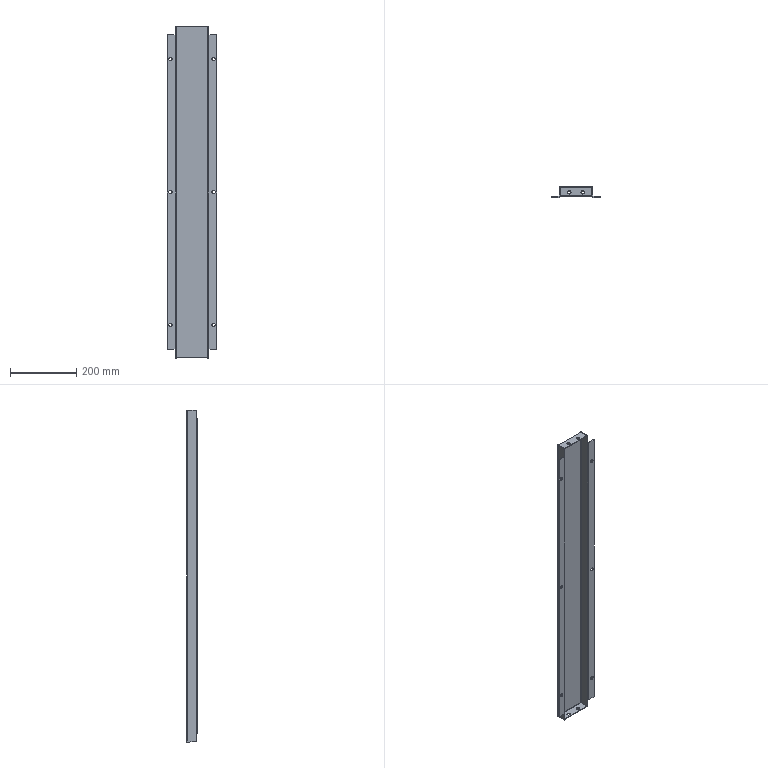Component | SolidWorks | 19MiddleUpperBeam-1 | 1 solid | 82 faces | volume 415370 mm3 | plane 50 | cylinder 32 | commonest cylinder face diameters 10 x20 6 x6 2 x6